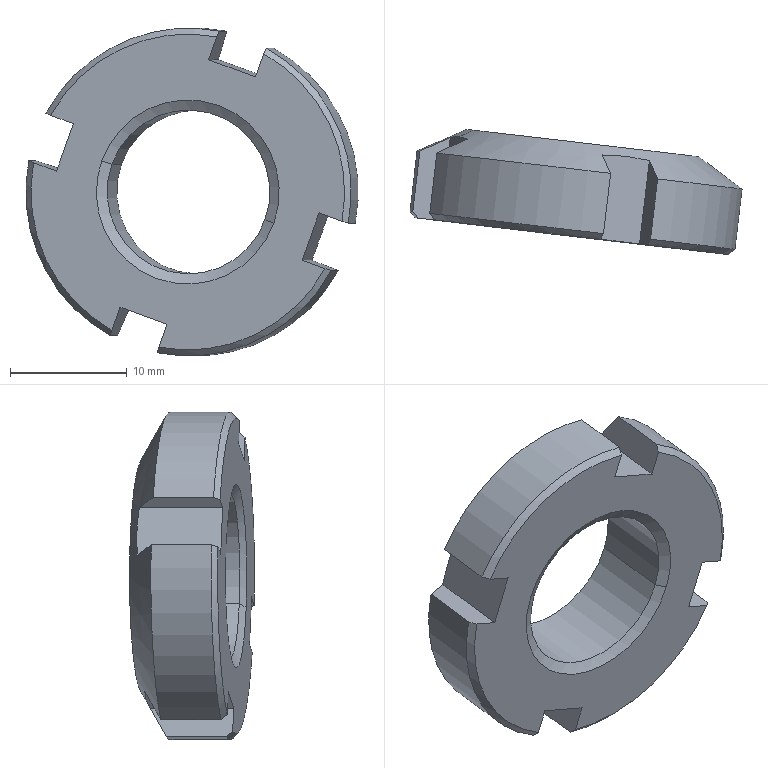Component | SolidWorks | 8TC-A17001-91-00UpperAndLowerPressAssembly-1_GB812RoundNutM14_1.5-1 | 1 solid | 30 faces | box 28.41 x 10.69 x 28 mm | volume 2997 mm3 | plane 14 | cone 10 | cylinder 6 | commonest cylinder face diameters 28 x4 14 x2 | material A3
STEP:
#1=CARTESIAN_POINT('',(-0.3344,-4.257,-1.954));
#2=VERTEX_POINT('',#1);
#3=CARTESIAN_POINT('',(0.1805,-4.318,-2.141));
#4=VERTEX_POINT('',#3);
#5=CARTESIAN_POINT('',(-0.07696,-4.287,-2.047));
#6=DIRECTION('',(-0.1167,-0.9932,0.));
#7=DIRECTION('',(0.9342,-0.1097,-0.3394));
#8=AXIS2_PLACEMENT_3D('',#5,#6,#7);
#9=CIRCLE('',#8,0.2756);
#10=EDGE_CURVE('',#2,#4,#9,.T.);
#11=ORIENTED_EDGE('',*,*,#10,.F.);
#12=CARTESIAN_POINT('',(-0.3686,-4.273,-1.942));
#13=VERTEX_POINT('',#12);
#14=CARTESIAN_POINT('',(-0.3344,-4.257,-1.954));
#15=DIRECTION('',(-0.8674,-0.4016,0.2939));
#16=VECTOR('',#15,39.37);
#17=LINE('',#14,#16);
#18=EDGE_CURVE('',#2,#13,#17,.T.);
#19=ORIENTED_EDGE('',*,*,#18,.T.);
#20=CARTESIAN_POINT('',(0.2101,-4.341,-2.152));
#21=VERTEX_POINT('',#20);
#22=CARTESIAN_POINT('',(-0.07926,-4.307,-2.047));
#23=DIRECTION('',(0.1167,0.9932,-0.));
#24=DIRECTION('',(0.9342,-0.1097,-0.3394));
#25=AXIS2_PLACEMENT_3D('',#22,#23,#24);
#26=CIRCLE('',#25,0.3097);
#27=EDGE_CURVE('',#21,#13,#26,.T.);
#28=ORIENTED_EDGE('',*,*,#27,.F.);
#29=CARTESIAN_POINT('',(0.1805,-4.318,-2.141));
#30=DIRECTION('',(0.7507,-0.5916,-0.2939));
#31=VECTOR('',#30,39.37);
#32=LINE('',#29,#31);
#33=EDGE_CURVE('',#4,#21,#32,.T.);
#34=ORIENTED_EDGE('',*,*,#33,.F.);
#35=EDGE_LOOP('',(#11,#19,#28,#34));
#36=FACE_OUTER_BOUND('',#35,.T.);
#37=CARTESIAN_POINT('',(-0.07696,-4.287,-2.047));
#38=DIRECTION('',(-0.1167,-0.9932,0.));
#39=DIRECTION('',(0.9342,-0.1097,-0.3394));
#40=AXIS2_PLACEMENT_3D('',#37,#38,#39);
#41=CONICAL_SURFACE('',#40,0.2756,1.047);
#42=ADVANCED_FACE('',(#36),#41,.F.);
#43=CARTESIAN_POINT('',(0.2126,-4.044,-2.141));
#44=VERTEX_POINT('',#43);
#45=CARTESIAN_POINT('',(-0.3023,-3.983,-1.954));
#46=VERTEX_POINT('',#45);
#47=CARTESIAN_POINT('',(-0.04481,-4.014,-2.047));
#48=DIRECTION('',(0.1167,0.9932,-0.));
#49=DIRECTION('',(0.9342,-0.1097,-0.3394));
#50=AXIS2_PLACEMENT_3D('',#47,#48,#49);
#51=CIRCLE('',#50,0.2756);
#52=EDGE_CURVE('',#44,#46,#51,.T.);
#53=ORIENTED_EDGE('',*,*,#52,.F.);
#54=CARTESIAN_POINT('',(0.2468,-4.028,-2.152));
#55=VERTEX_POINT('',#54);
#56=CARTESIAN_POINT('',(0.2468,-4.028,-2.152));
#57=DIRECTION('',(0.8674,0.4016,-0.2939));
#58=VECTOR('',#57,39.37);
#59=LINE('',#56,#58);
#60=EDGE_CURVE('',#44,#55,#59,.T.);
#61=ORIENTED_EDGE('',*,*,#60,.T.);
#62=CARTESIAN_POINT('',(-0.3318,-3.96,-1.942));
#63=VERTEX_POINT('',#62);
#64=CARTESIAN_POINT('',(-0.04251,-3.994,-2.047));
#65=DIRECTION('',(-0.1167,-0.9932,0.));
#66=DIRECTION('',(0.9342,-0.1097,-0.3394));
#67=AXIS2_PLACEMENT_3D('',#64,#65,#66);
#68=CIRCLE('',#67,0.3097);
#69=EDGE_CURVE('',#63,#55,#68,.T.);
#70=ORIENTED_EDGE('',*,*,#69,.F.);
#71=CARTESIAN_POINT('',(-0.3318,-3.96,-1.942));
#72=DIRECTION('',(-0.7507,0.5916,0.2939));
#73=VECTOR('',#72,39.37);
#74=LINE('',#71,#73);
#75=EDGE_CURVE('',#46,#63,#74,.T.);
#76=ORIENTED_EDGE('',*,*,#75,.F.);
#77=EDGE_LOOP('',(#53,#61,#70,#76));
#78=FACE_OUTER_BOUND('',#77,.T.);
#79=CARTESIAN_POINT('',(-0.04251,-3.994,-2.047));
#80=DIRECTION('',(0.1167,0.9932,-0.));
#81=DIRECTION('',(-0.9342,0.1097,0.3394));
#82=AXIS2_PLACEMENT_3D('',#79,#80,#81);
#83=CONICAL_SURFACE('',#82,0.3097,1.047);
#84=ADVANCED_FACE('',(#78),#83,.F.);
#85=CARTESIAN_POINT('',(-0.4103,-3.951,-1.914));
#86=VERTEX_POINT('',#85);
#87=CARTESIAN_POINT('',(0.3253,-4.037,-2.181));
#88=VERTEX_POINT('',#87);
#89=CARTESIAN_POINT('',(-0.04251,-3.994,-2.047));
#90=DIRECTION('',(0.1167,0.9932,-0.));
#91=DIRECTION('',(0.9342,-0.1097,-0.3394));
#92=AXIS2_PLACEMENT_3D('',#89,#90,#91);
#93=CIRCLE('',#92,0.3937);
#94=EDGE_CURVE('',#86,#88,#93,.T.);
#95=ORIENTED_EDGE('',*,*,#94,.F.);
#96=CARTESIAN_POINT('',(-0.459,-3.973,-1.897));
#97=VERTEX_POINT('',#96);
#98=CARTESIAN_POINT('',(-0.568,-4.024,-1.86));
#99=DIRECTION('',(-0.8674,-0.4015,0.2939));
#100=VECTOR('',#99,39.37);
#101=LINE('',#98,#100);
#102=EDGE_CURVE('',#86,#97,#101,.T.);
#103=ORIENTED_EDGE('',*,*,#102,.T.);
#104=CARTESIAN_POINT('',(-0.431,-3.981,-1.818));
#105=VERTEX_POINT('',#104);
#106=CARTESIAN_POINT('',(-0.431,-3.981,-1.818));
#107=CARTESIAN_POINT('',(-0.4401,-3.977,-1.844));
#108=CARTESIAN_POINT('',(-0.4494,-3.974,-1.87));
#109=CARTESIAN_POINT('',(-0.459,-3.973,-1.897));
#110=B_SPLINE_CURVE_WITH_KNOTS('',3,(#106,#107,#108,#109),.UNSPECIFIED.,.F.,.F.,(4,4),(0.002413,0.004566),.UNSPECIFIED.);
#111=EDGE_CURVE('',#105,#97,#110,.T.);
#112=ORIENTED_EDGE('',*,*,#111,.F.);
#113=CARTESIAN_POINT('',(-0.5334,-4.028,-1.783));
#114=VERTEX_POINT('',#113);
#115=CARTESIAN_POINT('',(-0.5334,-4.028,-1.783));
#116=CARTESIAN_POINT('',(-0.4993,-4.012,-1.794));
#117=CARTESIAN_POINT('',(-0.4651,-3.997,-1.806));
#118=CARTESIAN_POINT('',(-0.431,-3.981,-1.818));
#119=B_SPLINE_CURVE_WITH_KNOTS('',3,(#115,#116,#117,#118),.UNSPECIFIED.,.F.,.F.,(4,4),(0.005991,0.008982),.UNSPECIFIED.);
#120=EDGE_CURVE('',#114,#105,#119,.T.);
#121=ORIENTED_EDGE('',*,*,#120,.F.);
#122=CARTESIAN_POINT('',(0.0514,-4.097,-1.506));
#123=VERTEX_POINT('',#122);
#124=CARTESIAN_POINT('',(-0.05312,-4.084,-2.047));
#125=DIRECTION('',(-0.1167,-0.9932,0.));
#126=DIRECTION('',(0.9342,-0.1097,-0.3394));
#127=AXIS2_PLACEMENT_3D('',#124,#125,#126);
#128=CIRCLE('',#127,0.5512);
#129=EDGE_CURVE('',#123,#114,#128,.T.);
#130=ORIENTED_EDGE('',*,*,#129,.F.);
#131=CARTESIAN_POINT('',(0.02368,-4.035,-1.602));
#132=VERTEX_POINT('',#131);
#133=CARTESIAN_POINT('',(0.02368,-4.035,-1.602));
#134=CARTESIAN_POINT('',(0.03294,-4.055,-1.57));
#135=CARTESIAN_POINT('',(0.04217,-4.076,-1.538));
#136=CARTESIAN_POINT('',(0.0514,-4.097,-1.506));
#137=B_SPLINE_CURVE_WITH_KNOTS('',3,(#133,#134,#135,#136),.UNSPECIFIED.,.F.,.F.,(4,4),(0.006116,0.009107),.UNSPECIFIED.);
#138=EDGE_CURVE('',#132,#123,#137,.T.);
#139=ORIENTED_EDGE('',*,*,#138,.F.);
#140=CARTESIAN_POINT('',(0.1818,-4.053,-1.66));
#141=VERTEX_POINT('',#140);
#142=CARTESIAN_POINT('',(0.1818,-4.053,-1.66));
#143=CARTESIAN_POINT('',(0.156,-4.047,-1.65));
#144=CARTESIAN_POINT('',(0.1299,-4.043,-1.641));
#145=CARTESIAN_POINT('',(0.09038,-4.038,-1.627));
#146=CARTESIAN_POINT('',(0.07712,-4.037,-1.622));
#147=CARTESIAN_POINT('',(0.05046,-4.035,-1.612));
#148=CARTESIAN_POINT('',(0.03703,-4.035,-1.607));
#149=CARTESIAN_POINT('',(0.02368,-4.035,-1.602));
#150=B_SPLINE_CURVE_WITH_KNOTS('',3,(#142,#143,#144,#145,#146,#147,#148,#149),.UNSPECIFIED.,.F.,.F.,(4,2,2,4),(0.002413,0.004558,0.005631,0.006704),.UNSPECIFIED.);
#151=EDGE_CURVE('',#141,#132,#150,.T.);
#152=ORIENTED_EDGE('',*,*,#151,.F.);
#153=CARTESIAN_POINT('',(0.2096,-4.115,-1.564));
#154=VERTEX_POINT('',#153);
#155=CARTESIAN_POINT('',(0.2096,-4.115,-1.564));
#156=CARTESIAN_POINT('',(0.2003,-4.095,-1.596));
#157=CARTESIAN_POINT('',(0.1911,-4.074,-1.628));
#158=CARTESIAN_POINT('',(0.1818,-4.053,-1.66));
#159=B_SPLINE_CURVE_WITH_KNOTS('',3,(#155,#156,#157,#158),.UNSPECIFIED.,.F.,.F.,(4,4),(0.003725,0.006717),.UNSPECIFIED.);
#160=EDGE_CURVE('',#154,#141,#159,.T.);
#161=ORIENTED_EDGE('',*,*,#160,.F.);
#162=CARTESIAN_POINT('',(0.4842,-4.147,-2.152));
#163=VERTEX_POINT('',#162);
#164=CARTESIAN_POINT('',(-0.05312,-4.084,-2.047));
#165=DIRECTION('',(-0.1167,-0.9932,0.));
#166=DIRECTION('',(0.9342,-0.1097,-0.3394));
#167=AXIS2_PLACEMENT_3D('',#164,#165,#166);
#168=CIRCLE('',#167,0.5512);
#169=EDGE_CURVE('',#163,#154,#168,.T.);
#170=ORIENTED_EDGE('',*,*,#169,.F.);
#171=CARTESIAN_POINT('',(0.3954,-4.078,-2.118));
#172=VERTEX_POINT('',#171);
#173=CARTESIAN_POINT('',(0.3954,-4.078,-2.118));
#174=CARTESIAN_POINT('',(0.425,-4.101,-2.129));
#175=CARTESIAN_POINT('',(0.4546,-4.124,-2.141));
#176=CARTESIAN_POINT('',(0.4842,-4.147,-2.152));
#177=B_SPLINE_CURVE_WITH_KNOTS('',3,(#173,#174,#175,#176),.UNSPECIFIED.,.F.,.F.,(4,4),(0.006116,0.009107),.UNSPECIFIED.);
#178=EDGE_CURVE('',#172,#163,#177,.T.);
#179=ORIENTED_EDGE('',*,*,#178,.F.);
#180=CARTESIAN_POINT('',(0.3674,-4.07,-2.197));
#181=VERTEX_POINT('',#180);
#182=CARTESIAN_POINT('',(0.3674,-4.07,-2.197));
#183=CARTESIAN_POINT('',(0.3769,-4.072,-2.171));
#184=CARTESIAN_POINT('',(0.3863,-4.074,-2.144));
#185=CARTESIAN_POINT('',(0.3954,-4.078,-2.118));
#186=B_SPLINE_CURVE_WITH_KNOTS('',3,(#182,#183,#184,#185),.UNSPECIFIED.,.F.,.F.,(4,4),(0.01138,0.01353),.UNSPECIFIED.);
#187=EDGE_CURVE('',#181,#172,#186,.T.);
#188=ORIENTED_EDGE('',*,*,#187,.F.);
#189=CARTESIAN_POINT('',(0.4618,-4.145,-2.234));
#190=DIRECTION('',(0.7507,-0.5916,-0.2939));
#191=VECTOR('',#190,39.37);
#192=LINE('',#189,#191);
#193=EDGE_CURVE('',#88,#181,#192,.T.);
#194=ORIENTED_EDGE('',*,*,#193,.F.);
#195=EDGE_LOOP('',(#95,#103,#112,#121,#130,#139,#152,#161,#170,#179,#188,#194));
#196=FACE_OUTER_BOUND('',#195,.T.);
#197=CARTESIAN_POINT('',(-0.05312,-4.084,-2.047));
#198=DIRECTION('',(-0.1167,-0.9932,0.));
#199=DIRECTION('',(0.9342,-0.1097,-0.3394));
#200=AXIS2_PLACEMENT_3D('',#197,#198,#199);
#201=CONICAL_SURFACE('',#200,0.5512,1.047);
#202=ADVANCED_FACE('',(#196),#201,.T.);
#203=ORIENTED_EDGE('',*,*,#10,.T.);
#204=CARTESIAN_POINT('',(0.1782,-4.337,-2.141));
#205=DIRECTION('',(0.1167,0.9932,-0.));
#206=VECTOR('',#205,39.37);
#207=LINE('',#204,#206);
#208=EDGE_CURVE('',#4,#44,#207,.T.);
#209=ORIENTED_EDGE('',*,*,#208,.T.);
#210=ORIENTED_EDGE('',*,*,#52,.T.);
#211=CARTESIAN_POINT('',(-0.3367,-4.277,-1.954));
#212=DIRECTION('',(0.1167,0.9932,-0.));
#213=VECTOR('',#212,39.37);
#214=LINE('',#211,#213);
#215=EDGE_CURVE('',#2,#46,#214,.T.);
#216=ORIENTED_EDGE('',*,*,#215,.F.);
#217=EDGE_LOOP('',(#203,#209,#210,#216));
#218=FACE_OUTER_BOUND('',#217,.T.);
#219=CARTESIAN_POINT('',(-0.07926,-4.307,-2.047));
#220=DIRECTION('',(0.1167,0.9932,-0.));
#221=DIRECTION('',(-0.9342,0.1097,0.3394));
#222=AXIS2_PLACEMENT_3D('',#219,#220,#221);
#223=CYLINDRICAL_SURFACE('',#222,0.2756);
#224=ADVANCED_FACE('',(#218),#223,.F.);
#225=CARTESIAN_POINT('',(0.1857,-4.318,-1.564));
#226=VERTEX_POINT('',#225);
#227=CARTESIAN_POINT('',(0.4604,-4.35,-2.152));
#228=VERTEX_POINT('',#227);
#229=CARTESIAN_POINT('',(-0.07696,-4.287,-2.047));
#230=DIRECTION('',(0.1167,0.9932,-0.));
#231=DIRECTION('',(0.9342,-0.1097,-0.3394));
#232=AXIS2_PLACEMENT_3D('',#229,#230,#231);
#233=CIRCLE('',#232,0.5512);
#234=EDGE_CURVE('',#226,#228,#233,.T.);
#235=ORIENTED_EDGE('',*,*,#234,.T.);
#236=CARTESIAN_POINT('',(0.4948,-4.057,-2.152));
#237=DIRECTION('',(-0.1167,-0.9932,0.));
#238=VECTOR('',#237,39.37);
#239=LINE('',#236,#238);
#240=EDGE_CURVE('',#163,#228,#239,.T.);
#241=ORIENTED_EDGE('',*,*,#240,.F.);
#242=ORIENTED_EDGE('',*,*,#169,.T.);
#243=CARTESIAN_POINT('',(0.2202,-4.025,-1.564));
#244=DIRECTION('',(-0.1167,-0.9932,0.));
#245=VECTOR('',#244,39.37);
#246=LINE('',#243,#245);
#247=EDGE_CURVE('',#154,#226,#246,.T.);
#248=ORIENTED_EDGE('',*,*,#247,.T.);
#249=EDGE_LOOP('',(#235,#241,#242,#248));
#250=FACE_OUTER_BOUND('',#249,.T.);
#251=CARTESIAN_POINT('',(-0.07926,-4.307,-2.047));
#252=DIRECTION('',(0.1167,0.9932,-0.));
#253=DIRECTION('',(-0.9342,0.1097,0.3394));
#254=AXIS2_PLACEMENT_3D('',#251,#252,#253);
#255=CYLINDRICAL_SURFACE('',#254,0.5512);
#256=ADVANCED_FACE('',(#250),#255,.T.);
#257=CARTESIAN_POINT('',(0.4395,-4.368,-2.146));
#258=VERTEX_POINT('',#257);
#259=CARTESIAN_POINT('',(0.4604,-4.35,-2.152));
#260=CARTESIAN_POINT('',(0.4534,-4.356,-2.15));
#261=CARTESIAN_POINT('',(0.4464,-4.362,-2.148));
#262=CARTESIAN_POINT('',(0.4395,-4.368,-2.146));
#263=B_SPLINE_CURVE_WITH_KNOTS('',3,(#259,#260,#261,#262),.UNSPECIFIED.,.F.,.F.,(4,4),(0.004508,0.005219),.UNSPECIFIED.);
#264=EDGE_CURVE('',#228,#258,#263,.T.);
#265=ORIENTED_EDGE('',*,*,#264,.F.);
#266=ORIENTED_EDGE('',*,*,#234,.F.);
#267=CARTESIAN_POINT('',(0.1767,-4.337,-1.582));
#268=VERTEX_POINT('',#267);
#269=CARTESIAN_POINT('',(0.1767,-4.337,-1.582));
#270=CARTESIAN_POINT('',(0.1797,-4.331,-1.576));
#271=CARTESIAN_POINT('',(0.1827,-4.324,-1.57));
#272=CARTESIAN_POINT('',(0.1857,-4.318,-1.564));
#273=B_SPLINE_CURVE_WITH_KNOTS('',3,(#269,#270,#271,#272),.UNSPECIFIED.,.F.,.F.,(4,4),(0.00461,0.005321),.UNSPECIFIED.);
#274=EDGE_CURVE('',#268,#226,#273,.T.);
#275=ORIENTED_EDGE('',*,*,#274,.F.);
#276=CARTESIAN_POINT('',(-0.07926,-4.307,-2.047));
#277=DIRECTION('',(-0.1167,-0.9932,0.));
#278=DIRECTION('',(0.9342,-0.1097,-0.3394));
#279=AXIS2_PLACEMENT_3D('',#276,#277,#278);
#280=CIRCLE('',#279,0.5315);
#281=EDGE_CURVE('',#258,#268,#280,.T.);
#282=ORIENTED_EDGE('',*,*,#281,.F.);
#283=EDGE_LOOP('',(#265,#266,#275,#282));
#284=FACE_OUTER_BOUND('',#283,.T.);
#285=CARTESIAN_POINT('',(-0.07926,-4.307,-2.047));
#286=DIRECTION('',(0.1167,0.9932,-0.));
#287=DIRECTION('',(-0.9342,0.1097,0.3394));
#288=AXIS2_PLACEMENT_3D('',#285,#286,#287);
#289=CONICAL_SURFACE('',#288,0.5315,0.7854);
#290=ADVANCED_FACE('',(#284),#289,.T.);
#291=CARTESIAN_POINT('',(-0.5572,-4.231,-1.783));
#292=VERTEX_POINT('',#291);
#293=CARTESIAN_POINT('',(0.02755,-4.3,-1.506));
#294=VERTEX_POINT('',#293);
#295=CARTESIAN_POINT('',(-0.07696,-4.287,-2.047));
#296=DIRECTION('',(0.1167,0.9932,-0.));
#297=DIRECTION('',(0.9342,-0.1097,-0.3394));
#298=AXIS2_PLACEMENT_3D('',#295,#296,#297);
#299=CIRCLE('',#298,0.5512);
#300=EDGE_CURVE('',#292,#294,#299,.T.);
#301=ORIENTED_EDGE('',*,*,#300,.T.);
#302=CARTESIAN_POINT('',(0.062,-4.006,-1.506));
#303=DIRECTION('',(-0.1167,-0.9932,0.));
#304=VECTOR('',#303,39.37);
#305=LINE('',#302,#304);
#306=EDGE_CURVE('',#123,#294,#305,.T.);
#307=ORIENTED_EDGE('',*,*,#306,.F.);
#308=ORIENTED_EDGE('',*,*,#129,.T.);
#309=CARTESIAN_POINT('',(-0.5228,-3.938,-1.783));
#310=DIRECTION('',(-0.1167,-0.9932,0.));
#311=VECTOR('',#310,39.37);
#312=LINE('',#309,#311);
#313=EDGE_CURVE('',#114,#292,#312,.T.);
#314=ORIENTED_EDGE('',*,*,#313,.T.);
#315=EDGE_LOOP('',(#301,#307,#308,#314));
#316=FACE_OUTER_BOUND('',#315,.T.);
#317=CARTESIAN_POINT('',(-0.07926,-4.307,-2.047));
#318=DIRECTION('',(0.1167,0.9932,-0.));
#319=DIRECTION('',(-0.9342,0.1097,0.3394));
#320=AXIS2_PLACEMENT_3D('',#317,#318,#319);
#321=CYLINDRICAL_SURFACE('',#320,0.5512);
#322=ADVANCED_FACE('',(#316),#321,.T.);
#323=CARTESIAN_POINT('',(0.01854,-4.318,-1.525));
#324=VERTEX_POINT('',#323);
#325=CARTESIAN_POINT('',(0.02755,-4.3,-1.506));
#326=CARTESIAN_POINT('',(0.02455,-4.306,-1.512));
#327=CARTESIAN_POINT('',(0.02154,-4.312,-1.519));
#328=CARTESIAN_POINT('',(0.01854,-4.318,-1.525));
#329=B_SPLINE_CURVE_WITH_KNOTS('',3,(#325,#326,#327,#328),.UNSPECIFIED.,.F.,.F.,(4,4),(0.004508,0.005219),.UNSPECIFIED.);
#330=EDGE_CURVE('',#294,#324,#329,.T.);
#331=ORIENTED_EDGE('',*,*,#330,.F.);
#332=ORIENTED_EDGE('',*,*,#300,.F.);
#333=CARTESIAN_POINT('',(-0.5409,-4.253,-1.79));
#334=VERTEX_POINT('',#333);
#335=CARTESIAN_POINT('',(-0.5409,-4.253,-1.79));
#336=CARTESIAN_POINT('',(-0.5464,-4.245,-1.787));
#337=CARTESIAN_POINT('',(-0.5518,-4.238,-1.785));
#338=CARTESIAN_POINT('',(-0.5572,-4.231,-1.783));
#339=B_SPLINE_CURVE_WITH_KNOTS('',3,(#335,#336,#337,#338),.UNSPECIFIED.,.F.,.F.,(4,4),(0.00461,0.005321),.UNSPECIFIED.);
#340=EDGE_CURVE('',#334,#292,#339,.T.);
#341=ORIENTED_EDGE('',*,*,#340,.F.);
#342=CARTESIAN_POINT('',(-0.07926,-4.307,-2.047));
#343=DIRECTION('',(-0.1167,-0.9932,0.));
#344=DIRECTION('',(0.9342,-0.1097,-0.3394));
#345=AXIS2_PLACEMENT_3D('',#342,#343,#344);
#346=CIRCLE('',#345,0.5315);
#347=EDGE_CURVE('',#324,#334,#346,.T.);
#348=ORIENTED_EDGE('',*,*,#347,.F.);
#349=EDGE_LOOP('',(#331,#332,#341,#348));
#350=FACE_OUTER_BOUND('',#349,.T.);
#351=CARTESIAN_POINT('',(-0.07926,-4.307,-2.047));
#352=DIRECTION('',(0.1167,0.9932,-0.));
#353=DIRECTION('',(-0.9342,0.1097,0.3394));
#354=AXIS2_PLACEMENT_3D('',#351,#352,#353);
#355=CONICAL_SURFACE('',#354,0.5315,0.7854);
#356=ADVANCED_FACE('',(#350),#355,.T.);
#357=CARTESIAN_POINT('',(-0.3396,-4.256,-2.531));
#358=VERTEX_POINT('',#357);
#359=CARTESIAN_POINT('',(-0.6143,-4.224,-1.942));
#360=VERTEX_POINT('',#359);
#361=CARTESIAN_POINT('',(-0.07696,-4.287,-2.047));
#362=DIRECTION('',(0.1167,0.9932,-0.));
#363=DIRECTION('',(0.9342,-0.1097,-0.3394));
#364=AXIS2_PLACEMENT_3D('',#361,#362,#363);
#365=CIRCLE('',#364,0.5512);
#366=EDGE_CURVE('',#358,#360,#365,.T.);
#367=ORIENTED_EDGE('',*,*,#366,.T.);
#368=CARTESIAN_POINT('',(-0.5905,-4.021,-1.942));
#369=VERTEX_POINT('',#368);
#370=CARTESIAN_POINT('',(-0.5799,-3.931,-1.942));
#371=DIRECTION('',(-0.1167,-0.9932,0.));
#372=VECTOR('',#371,39.37);
#373=LINE('',#370,#372);
#374=EDGE_CURVE('',#369,#360,#373,.T.);
#375=ORIENTED_EDGE('',*,*,#374,.F.);
#376=CARTESIAN_POINT('',(-0.3158,-4.053,-2.531));
#377=VERTEX_POINT('',#376);
#378=CARTESIAN_POINT('',(-0.05312,-4.084,-2.047));
#379=DIRECTION('',(-0.1167,-0.9932,0.));
#380=DIRECTION('',(0.9342,-0.1097,-0.3394));
#381=AXIS2_PLACEMENT_3D('',#378,#379,#380);
#382=CIRCLE('',#381,0.5512);
#383=EDGE_CURVE('',#369,#377,#382,.T.);
#384=ORIENTED_EDGE('',*,*,#383,.T.);
#385=CARTESIAN_POINT('',(-0.3052,-3.963,-2.531));
#386=DIRECTION('',(-0.1167,-0.9932,0.));
#387=VECTOR('',#386,39.37);
#388=LINE('',#385,#387);
#389=EDGE_CURVE('',#377,#358,#388,.T.);
#390=ORIENTED_EDGE('',*,*,#389,.T.);
#391=EDGE_LOOP('',(#367,#375,#384,#390));
#392=FACE_OUTER_BOUND('',#391,.T.);
#393=CARTESIAN_POINT('',(-0.07926,-4.307,-2.047));
#394=DIRECTION('',(0.1167,0.9932,-0.));
#395=DIRECTION('',(-0.9342,0.1097,0.3394));
#396=AXIS2_PLACEMENT_3D('',#393,#394,#395);
#397=CYLINDRICAL_SURFACE('',#396,0.5512);
#398=ADVANCED_FACE('',(#392),#397,.T.);
#399=CARTESIAN_POINT('',(-0.598,-4.246,-1.949));
#400=VERTEX_POINT('',#399);
#401=CARTESIAN_POINT('',(-0.6143,-4.224,-1.942));
#402=CARTESIAN_POINT('',(-0.6089,-4.231,-1.944));
#403=CARTESIAN_POINT('',(-0.6034,-4.239,-1.947));
#404=CARTESIAN_POINT('',(-0.598,-4.246,-1.949));
#405=B_SPLINE_CURVE_WITH_KNOTS('',3,(#401,#402,#403,#404),.UNSPECIFIED.,.F.,.F.,(4,4),(0.004508,0.005219),.UNSPECIFIED.);
#406=EDGE_CURVE('',#360,#400,#405,.T.);
#407=ORIENTED_EDGE('',*,*,#406,.F.);
#408=ORIENTED_EDGE('',*,*,#366,.F.);
#409=CARTESIAN_POINT('',(-0.3352,-4.277,-2.512));
#410=VERTEX_POINT('',#409);
#411=CARTESIAN_POINT('',(-0.3352,-4.277,-2.512));
#412=CARTESIAN_POINT('',(-0.3367,-4.27,-2.518));
#413=CARTESIAN_POINT('',(-0.3382,-4.263,-2.525));
#414=CARTESIAN_POINT('',(-0.3396,-4.256,-2.531));
#415=B_SPLINE_CURVE_WITH_KNOTS('',3,(#411,#412,#413,#414),.UNSPECIFIED.,.F.,.F.,(4,4),(0.00461,0.005321),.UNSPECIFIED.);
#416=EDGE_CURVE('',#410,#358,#415,.T.);
#417=ORIENTED_EDGE('',*,*,#416,.F.);
#418=CARTESIAN_POINT('',(-0.07926,-4.307,-2.047));
#419=DIRECTION('',(-0.1167,-0.9932,0.));
#420=DIRECTION('',(0.9342,-0.1097,-0.3394));
#421=AXIS2_PLACEMENT_3D('',#418,#419,#420);
#422=CIRCLE('',#421,0.5315);
#423=EDGE_CURVE('',#400,#410,#422,.T.);
#424=ORIENTED_EDGE('',*,*,#423,.F.);
#425=EDGE_LOOP('',(#407,#408,#417,#424));
#426=FACE_OUTER_BOUND('',#425,.T.);
#427=CARTESIAN_POINT('',(-0.07926,-4.307,-2.047));
#428=DIRECTION('',(0.1167,0.9932,-0.));
#429=DIRECTION('',(-0.9342,0.1097,0.3394));
#430=AXIS2_PLACEMENT_3D('',#427,#428,#429);
#431=CONICAL_SURFACE('',#430,0.5315,0.7854);
#432=ADVANCED_FACE('',(#426),#431,.T.);
#433=ORIENTED_EDGE('',*,*,#27,.T.);
#434=CARTESIAN_POINT('',(-0.07926,-4.307,-2.047));
#435=DIRECTION('',(0.1167,0.9932,-0.));
#436=DIRECTION('',(0.9342,-0.1097,-0.3394));
#437=AXIS2_PLACEMENT_3D('',#434,#435,#436);
#438=CIRCLE('',#437,0.3097);
#439=EDGE_CURVE('',#13,#21,#438,.T.);
#440=ORIENTED_EDGE('',*,*,#439,.T.);
#441=EDGE_LOOP('',(#433,#440));
#442=FACE_BOUND('',#441,.T.);
#443=CARTESIAN_POINT('',(0.3625,-4.359,-2.118));
#444=VERTEX_POINT('',#443);
#445=CARTESIAN_POINT('',(0.3625,-4.359,-2.118));
#446=DIRECTION('',(-0.9342,0.1097,0.3394));
#447=VECTOR('',#446,39.37);
#448=LINE('',#445,#447);
#449=EDGE_CURVE('',#258,#444,#448,.T.);
#450=ORIENTED_EDGE('',*,*,#449,.F.);
#451=ORIENTED_EDGE('',*,*,#281,.T.);
#452=CARTESIAN_POINT('',(0.1489,-4.334,-1.66));
#453=VERTEX_POINT('',#452);
#454=CARTESIAN_POINT('',(0.1489,-4.334,-1.66));
#455=DIRECTION('',(0.3371,-0.0396,0.9406));
#456=VECTOR('',#455,39.37);
#457=LINE('',#454,#456);
#458=EDGE_CURVE('',#453,#268,#457,.T.);
#459=ORIENTED_EDGE('',*,*,#458,.F.);
#460=CARTESIAN_POINT('',(-0.009248,-4.315,-1.602));
#461=VERTEX_POINT('',#460);
#462=CARTESIAN_POINT('',(0.1489,-4.334,-1.66));
#463=DIRECTION('',(0.9342,-0.1097,-0.3394));
#464=VECTOR('',#463,39.37);
#465=LINE('',#462,#464);
#466=EDGE_CURVE('',#461,#453,#465,.T.);
#467=ORIENTED_EDGE('',*,*,#466,.F.);
#468=CARTESIAN_POINT('',(-0.009248,-4.315,-1.602));
#469=DIRECTION('',(-0.3371,0.0396,-0.9406));
#470=VECTOR('',#469,39.37);
#471=LINE('',#468,#470);
#472=EDGE_CURVE('',#324,#461,#471,.T.);
#473=ORIENTED_EDGE('',*,*,#472,.F.);
#474=ORIENTED_EDGE('',*,*,#347,.T.);
#475=CARTESIAN_POINT('',(-0.4639,-4.262,-1.818));
#476=VERTEX_POINT('',#475);
#477=CARTESIAN_POINT('',(-0.4639,-4.262,-1.818));
#478=DIRECTION('',(-0.9342,0.1097,0.3394));
#479=VECTOR('',#478,39.37);
#480=LINE('',#477,#479);
#481=EDGE_CURVE('',#476,#334,#480,.T.);
#482=ORIENTED_EDGE('',*,*,#481,.F.);
#483=CARTESIAN_POINT('',(-0.521,-4.255,-1.977));
#484=VERTEX_POINT('',#483);
#485=CARTESIAN_POINT('',(-0.4639,-4.262,-1.818));
#486=DIRECTION('',(0.3371,-0.0396,0.9406));
#487=VECTOR('',#486,39.37);
#488=LINE('',#485,#487);
#489=EDGE_CURVE('',#484,#476,#488,.T.);
#490=ORIENTED_EDGE('',*,*,#489,.F.);
#491=CARTESIAN_POINT('',(-0.521,-4.255,-1.977));
#492=DIRECTION('',(0.9342,-0.1097,-0.3394));
#493=VECTOR('',#492,39.37);
#494=LINE('',#491,#493);
#495=EDGE_CURVE('',#400,#484,#494,.T.);
#496=ORIENTED_EDGE('',*,*,#495,.F.);
#497=ORIENTED_EDGE('',*,*,#423,.T.);
#498=CARTESIAN_POINT('',(-0.3074,-4.28,-2.435));
#499=VERTEX_POINT('',#498);
#500=CARTESIAN_POINT('',(-0.3074,-4.28,-2.435));
#501=DIRECTION('',(-0.3371,0.0396,-0.9406));
#502=VECTOR('',#501,39.37);
#503=LINE('',#500,#502);
#504=EDGE_CURVE('',#499,#410,#503,.T.);
#505=ORIENTED_EDGE('',*,*,#504,.F.);
#506=CARTESIAN_POINT('',(-0.1493,-4.299,-2.492));
#507=VERTEX_POINT('',#506);
#508=CARTESIAN_POINT('',(-0.3074,-4.28,-2.435));
#509=DIRECTION('',(-0.9342,0.1097,0.3394));
#510=VECTOR('',#509,39.37);
#511=LINE('',#508,#510);
#512=EDGE_CURVE('',#507,#499,#511,.T.);
#513=ORIENTED_EDGE('',*,*,#512,.F.);
#514=CARTESIAN_POINT('',(-0.1771,-4.295,-2.57));
#515=VERTEX_POINT('',#514);
#516=CARTESIAN_POINT('',(-0.1493,-4.299,-2.492));
#517=DIRECTION('',(0.3371,-0.0396,0.9406));
#518=VECTOR('',#517,39.37);
#519=LINE('',#516,#518);
#520=EDGE_CURVE('',#515,#507,#519,.T.);
#521=ORIENTED_EDGE('',*,*,#520,.F.);
#522=CARTESIAN_POINT('',(0.3824,-4.361,-2.305));
#523=VERTEX_POINT('',#522);
#524=CARTESIAN_POINT('',(-0.07926,-4.307,-2.047));
#525=DIRECTION('',(-0.1167,-0.9932,0.));
#526=DIRECTION('',(0.9342,-0.1097,-0.3394));
#527=AXIS2_PLACEMENT_3D('',#524,#525,#526);
#528=CIRCLE('',#527,0.5315);
#529=EDGE_CURVE('',#515,#523,#528,.T.);
#530=ORIENTED_EDGE('',*,*,#529,.T.);
#531=CARTESIAN_POINT('',(0.3054,-4.352,-2.277));
#532=VERTEX_POINT('',#531);
#533=CARTESIAN_POINT('',(0.3054,-4.352,-2.277));
#534=DIRECTION('',(0.9342,-0.1097,-0.3394));
#535=VECTOR('',#534,39.37);
#536=LINE('',#533,#535);
#537=EDGE_CURVE('',#532,#523,#536,.T.);
#538=ORIENTED_EDGE('',*,*,#537,.F.);
#539=CARTESIAN_POINT('',(0.3054,-4.352,-2.277));
#540=DIRECTION('',(-0.3371,0.0396,-0.9406));
#541=VECTOR('',#540,39.37);
#542=LINE('',#539,#541);
#543=EDGE_CURVE('',#444,#532,#542,.T.);
#544=ORIENTED_EDGE('',*,*,#543,.F.);
#545=EDGE_LOOP('',(#450,#451,#459,#467,#473,#474,#482,#490,#496,#497,#505,#513,#521,#530,#538,#544));
#546=FACE_OUTER_BOUND('',#545,.T.);
#547=CARTESIAN_POINT('',(-0.07926,-4.307,-2.047));
#548=DIRECTION('',(-0.1167,-0.9932,0.));
#549=DIRECTION('',(0.9342,-0.1097,-0.3394));
#550=AXIS2_PLACEMENT_3D('',#547,#548,#549);
#551=PLANE('',#550);
#552=ADVANCED_FACE('',(#442,#546),#551,.T.);
#553=ORIENTED_EDGE('',*,*,#69,.T.);
#554=CARTESIAN_POINT('',(-0.04251,-3.994,-2.047));
#555=DIRECTION('',(-0.1167,-0.9932,0.));
#556=DIRECTION('',(0.9342,-0.1097,-0.3394));
#557=AXIS2_PLACEMENT_3D('',#554,#555,#556);
#558=CIRCLE('',#557,0.3097);
#559=EDGE_CURVE('',#55,#63,#558,.T.);
#560=ORIENTED_EDGE('',*,*,#559,.T.);
#561=EDGE_LOOP('',(#553,#560));
#562=FACE_BOUND('',#561,.T.);
#563=CARTESIAN_POINT('',(-0.04251,-3.994,-2.047));
#564=DIRECTION('',(0.1167,0.9932,-0.));
#565=DIRECTION('',(0.9342,-0.1097,-0.3394));
#566=AXIS2_PLACEMENT_3D('',#563,#564,#565);
#567=CIRCLE('',#566,0.3937);
#568=EDGE_CURVE('',#88,#86,#567,.T.);
#569=ORIENTED_EDGE('',*,*,#568,.T.);
#570=ORIENTED_EDGE('',*,*,#94,.T.);
#571=EDGE_LOOP('',(#569,#570));
#572=FACE_OUTER_BOUND('',#571,.T.);
#573=CARTESIAN_POINT('',(-0.04251,-3.994,-2.047));
#574=DIRECTION('',(-0.1167,-0.9932,0.));
#575=DIRECTION('',(0.9342,-0.1097,-0.3394));
#576=AXIS2_PLACEMENT_3D('',#573,#574,#575);
#577=PLANE('',#576);
#578=ADVANCED_FACE('',(#562,#572),#577,.F.);
#579=CARTESIAN_POINT('',(-0.1576,-4.072,-2.588));
#580=VERTEX_POINT('',#579);
#581=CARTESIAN_POINT('',(0.4272,-4.141,-2.312));
#582=VERTEX_POINT('',#581);
#583=CARTESIAN_POINT('',(-0.05312,-4.084,-2.047));
#584=DIRECTION('',(-0.1167,-0.9932,0.));
#585=DIRECTION('',(0.9342,-0.1097,-0.3394));
#586=AXIS2_PLACEMENT_3D('',#583,#584,#585);
#587=CIRCLE('',#586,0.5512);
#588=EDGE_CURVE('',#580,#582,#587,.T.);
#589=ORIENTED_EDGE('',*,*,#588,.T.);
#590=CARTESIAN_POINT('',(0.4033,-4.344,-2.312));
#591=VERTEX_POINT('',#590);
#592=CARTESIAN_POINT('',(0.4378,-4.05,-2.312));
#593=DIRECTION('',(-0.1167,-0.9932,0.));
#594=VECTOR('',#593,39.37);
#595=LINE('',#592,#594);
#596=EDGE_CURVE('',#582,#591,#595,.T.);
#597=ORIENTED_EDGE('',*,*,#596,.T.);
#598=CARTESIAN_POINT('',(-0.1815,-4.275,-2.588));
#599=VERTEX_POINT('',#598);
#600=CARTESIAN_POINT('',(-0.07696,-4.287,-2.047));
#601=DIRECTION('',(0.1167,0.9932,-0.));
#602=DIRECTION('',(0.9342,-0.1097,-0.3394));
#603=AXIS2_PLACEMENT_3D('',#600,#601,#602);
#604=CIRCLE('',#603,0.5512);
#605=EDGE_CURVE('',#591,#599,#604,.T.);
#606=ORIENTED_EDGE('',*,*,#605,.T.);
#607=CARTESIAN_POINT('',(-0.147,-3.982,-2.588));
#608=DIRECTION('',(-0.1167,-0.9932,0.));
#609=VECTOR('',#608,39.37);
#610=LINE('',#607,#609);
#611=EDGE_CURVE('',#580,#599,#610,.T.);
#612=ORIENTED_EDGE('',*,*,#611,.F.);
#613=EDGE_LOOP('',(#589,#597,#606,#612));
#614=FACE_OUTER_BOUND('',#613,.T.);
#615=CARTESIAN_POINT('',(-0.07926,-4.307,-2.047));
#616=DIRECTION('',(0.1167,0.9932,-0.));
#617=DIRECTION('',(-0.9342,0.1097,0.3394));
#618=AXIS2_PLACEMENT_3D('',#615,#616,#617);
#619=CYLINDRICAL_SURFACE('',#618,0.5512);
#620=ADVANCED_FACE('',(#614),#619,.T.);
#621=ORIENTED_EDGE('',*,*,#208,.F.);
#622=CARTESIAN_POINT('',(-0.07696,-4.287,-2.047));
#623=DIRECTION('',(-0.1167,-0.9932,0.));
#624=DIRECTION('',(0.9342,-0.1097,-0.3394));
#625=AXIS2_PLACEMENT_3D('',#622,#623,#624);
#626=CIRCLE('',#625,0.2756);
#627=EDGE_CURVE('',#4,#2,#626,.T.);
#628=ORIENTED_EDGE('',*,*,#627,.T.);
#629=ORIENTED_EDGE('',*,*,#215,.T.);
#630=CARTESIAN_POINT('',(-0.04481,-4.014,-2.047));
#631=DIRECTION('',(0.1167,0.9932,-0.));
#632=DIRECTION('',(0.9342,-0.1097,-0.3394));
#633=AXIS2_PLACEMENT_3D('',#630,#631,#632);
#634=CIRCLE('',#633,0.2756);
#635=EDGE_CURVE('',#46,#44,#634,.T.);
#636=ORIENTED_EDGE('',*,*,#635,.T.);
#637=EDGE_LOOP('',(#621,#628,#629,#636));
#638=FACE_OUTER_BOUND('',#637,.T.);
#639=CARTESIAN_POINT('',(-0.07926,-4.307,-2.047));
#640=DIRECTION('',(0.1167,0.9932,-0.));
#641=DIRECTION('',(-0.9342,0.1097,0.3394));
#642=AXIS2_PLACEMENT_3D('',#639,#640,#641);
#643=CYLINDRICAL_SURFACE('',#642,0.2756);
#644=ADVANCED_FACE('',(#638),#643,.F.);
#645=CARTESIAN_POINT('',(0.3824,-4.361,-2.305));
#646=CARTESIAN_POINT('',(0.3894,-4.355,-2.307));
#647=CARTESIAN_POINT('',(0.3963,-4.35,-2.309));
#648=CARTESIAN_POINT('',(0.4033,-4.344,-2.312));
#649=B_SPLINE_CURVE_WITH_KNOTS('',3,(#645,#646,#647,#648),.UNSPECIFIED.,.F.,.F.,(4,4),(0.00461,0.005321),.UNSPECIFIED.);
#650=EDGE_CURVE('',#523,#591,#649,.T.);
#651=ORIENTED_EDGE('',*,*,#650,.F.);
#652=ORIENTED_EDGE('',*,*,#529,.F.);
#653=CARTESIAN_POINT('',(-0.1815,-4.275,-2.588));
#654=CARTESIAN_POINT('',(-0.18,-4.282,-2.582));
#655=CARTESIAN_POINT('',(-0.1785,-4.289,-2.576));
#656=CARTESIAN_POINT('',(-0.1771,-4.295,-2.57));
#657=B_SPLINE_CURVE_WITH_KNOTS('',3,(#653,#654,#655,#656),.UNSPECIFIED.,.F.,.F.,(4,4),(0.004508,0.005219),.UNSPECIFIED.);
#658=EDGE_CURVE('',#599,#515,#657,.T.);
#659=ORIENTED_EDGE('',*,*,#658,.F.);
#660=ORIENTED_EDGE('',*,*,#605,.F.);
#661=EDGE_LOOP('',(#651,#652,#659,#660));
#662=FACE_OUTER_BOUND('',#661,.T.);
#663=CARTESIAN_POINT('',(-0.07926,-4.307,-2.047));
#664=DIRECTION('',(0.1167,0.9932,-0.));
#665=DIRECTION('',(-0.9342,0.1097,0.3394));
#666=AXIS2_PLACEMENT_3D('',#663,#664,#665);
#667=CONICAL_SURFACE('',#666,0.5315,0.7854);
#668=ADVANCED_FACE('',(#662),#667,.T.);
#669=ORIENTED_EDGE('',*,*,#102,.F.);
#670=ORIENTED_EDGE('',*,*,#568,.F.);
#671=ORIENTED_EDGE('',*,*,#193,.T.);
#672=CARTESIAN_POINT('',(0.3383,-4.072,-2.277));
#673=VERTEX_POINT('',#672);
#674=CARTESIAN_POINT('',(0.3383,-4.072,-2.277));
#675=CARTESIAN_POINT('',(0.3432,-4.071,-2.264));
#676=CARTESIAN_POINT('',(0.3482,-4.07,-2.25));
#677=CARTESIAN_POINT('',(0.3579,-4.07,-2.224));
#678=CARTESIAN_POINT('',(0.3627,-4.07,-2.211));
#679=CARTESIAN_POINT('',(0.3674,-4.07,-2.197));
#680=B_SPLINE_CURVE_WITH_KNOTS('',3,(#674,#675,#676,#677,#678,#679),.UNSPECIFIED.,.F.,.F.,(4,2,4),(0.009256,0.01032,0.01138),.UNSPECIFIED.);
#681=EDGE_CURVE('',#673,#181,#680,.T.);
#682=ORIENTED_EDGE('',*,*,#681,.F.);
#683=CARTESIAN_POINT('',(0.4272,-4.141,-2.312));
#684=CARTESIAN_POINT('',(0.3976,-4.118,-2.3));
#685=CARTESIAN_POINT('',(0.368,-4.095,-2.289));
#686=CARTESIAN_POINT('',(0.3383,-4.072,-2.277));
#687=B_SPLINE_CURVE_WITH_KNOTS('',3,(#683,#684,#685,#686),.UNSPECIFIED.,.F.,.F.,(4,4),(0.003725,0.006717),.UNSPECIFIED.);
#688=EDGE_CURVE('',#582,#673,#687,.T.);
#689=ORIENTED_EDGE('',*,*,#688,.F.);
#690=ORIENTED_EDGE('',*,*,#588,.F.);
#691=CARTESIAN_POINT('',(-0.1163,-4.018,-2.492));
#692=VERTEX_POINT('',#691);
#693=CARTESIAN_POINT('',(-0.1163,-4.018,-2.492));
#694=CARTESIAN_POINT('',(-0.1301,-4.036,-2.524));
#695=CARTESIAN_POINT('',(-0.1439,-4.054,-2.556));
#696=CARTESIAN_POINT('',(-0.1576,-4.072,-2.588));
#697=B_SPLINE_CURVE_WITH_KNOTS('',3,(#693,#694,#695,#696),.UNSPECIFIED.,.F.,.F.,(4,4),(0.00385,0.006842),.UNSPECIFIED.);
#698=EDGE_CURVE('',#692,#580,#697,.T.);
#699=ORIENTED_EDGE('',*,*,#698,.F.);
#700=CARTESIAN_POINT('',(-0.2745,-4.,-2.435));
#701=VERTEX_POINT('',#700);
#702=CARTESIAN_POINT('',(-0.2745,-4.,-2.435));
#703=CARTESIAN_POINT('',(-0.2611,-4.,-2.439));
#704=CARTESIAN_POINT('',(-0.2477,-4.,-2.444));
#705=CARTESIAN_POINT('',(-0.2211,-4.002,-2.454));
#706=CARTESIAN_POINT('',(-0.2078,-4.003,-2.459));
#707=CARTESIAN_POINT('',(-0.1682,-4.008,-2.473));
#708=CARTESIAN_POINT('',(-0.1422,-4.012,-2.482));
#709=CARTESIAN_POINT('',(-0.1163,-4.018,-2.492));
#710=B_SPLINE_CURVE_WITH_KNOTS('',3,(#702,#703,#704,#705,#706,#707,#708,#709),.UNSPECIFIED.,.F.,.F.,(4,2,2,4),(0.009256,0.01032,0.01139,0.01353),.UNSPECIFIED.);
#711=EDGE_CURVE('',#701,#692,#710,.T.);
#712=ORIENTED_EDGE('',*,*,#711,.F.);
#713=CARTESIAN_POINT('',(-0.3158,-4.053,-2.531));
#714=CARTESIAN_POINT('',(-0.302,-4.036,-2.499));
#715=CARTESIAN_POINT('',(-0.2883,-4.018,-2.467));
#716=CARTESIAN_POINT('',(-0.2745,-4.,-2.435));
#717=B_SPLINE_CURVE_WITH_KNOTS('',3,(#713,#714,#715,#716),.UNSPECIFIED.,.F.,.F.,(4,4),(0.005991,0.008982),.UNSPECIFIED.);
#718=EDGE_CURVE('',#377,#701,#717,.T.);
#719=ORIENTED_EDGE('',*,*,#718,.F.);
#720=ORIENTED_EDGE('',*,*,#383,.F.);
#721=CARTESIAN_POINT('',(-0.488,-3.975,-1.977));
#722=VERTEX_POINT('',#721);
#723=CARTESIAN_POINT('',(-0.488,-3.975,-1.977));
#724=CARTESIAN_POINT('',(-0.5222,-3.99,-1.965));
#725=CARTESIAN_POINT('',(-0.5563,-4.006,-1.954));
#726=CARTESIAN_POINT('',(-0.5905,-4.021,-1.942));
#727=B_SPLINE_CURVE_WITH_KNOTS('',3,(#723,#724,#725,#726),.UNSPECIFIED.,.F.,.F.,(4,4),(0.00385,0.006842),.UNSPECIFIED.);
#728=EDGE_CURVE('',#722,#369,#727,.T.);
#729=ORIENTED_EDGE('',*,*,#728,.F.);
#730=CARTESIAN_POINT('',(-0.459,-3.973,-1.897));
#731=CARTESIAN_POINT('',(-0.4637,-3.973,-1.91));
#732=CARTESIAN_POINT('',(-0.4685,-3.973,-1.924));
#733=CARTESIAN_POINT('',(-0.4782,-3.973,-1.95));
#734=CARTESIAN_POINT('',(-0.4831,-3.974,-1.964));
#735=CARTESIAN_POINT('',(-0.488,-3.975,-1.977));
#736=B_SPLINE_CURVE_WITH_KNOTS('',3,(#730,#731,#732,#733,#734,#735),.UNSPECIFIED.,.F.,.F.,(4,2,4),(0.004566,0.005635,0.006704),.UNSPECIFIED.);
#737=EDGE_CURVE('',#97,#722,#736,.T.);
#738=ORIENTED_EDGE('',*,*,#737,.F.);
#739=EDGE_LOOP('',(#669,#670,#671,#682,#689,#690,#699,#712,#719,#720,#729,#738));
#740=FACE_OUTER_BOUND('',#739,.T.);
#741=CARTESIAN_POINT('',(-0.05312,-4.084,-2.047));
#742=DIRECTION('',(-0.1167,-0.9932,0.));
#743=DIRECTION('',(0.9342,-0.1097,-0.3394));
#744=AXIS2_PLACEMENT_3D('',#741,#742,#743);
#745=CONICAL_SURFACE('',#744,0.5512,1.047);
#746=ADVANCED_FACE('',(#740),#745,.T.);
#747=ORIENTED_EDGE('',*,*,#711,.T.);
#748=CARTESIAN_POINT('',(-0.1125,-3.986,-2.492));
#749=DIRECTION('',(-0.1167,-0.9932,0.));
#750=VECTOR('',#749,39.37);
#751=LINE('',#748,#750);
#752=EDGE_CURVE('',#692,#507,#751,.T.);
#753=ORIENTED_EDGE('',*,*,#752,.T.);
#754=ORIENTED_EDGE('',*,*,#512,.T.);
#755=CARTESIAN_POINT('',(-0.2707,-3.967,-2.435));
#756=DIRECTION('',(-0.1167,-0.9932,0.));
#757=VECTOR('',#756,39.37);
#758=LINE('',#755,#757);
#759=EDGE_CURVE('',#701,#499,#758,.T.);
#760=ORIENTED_EDGE('',*,*,#759,.F.);
#761=EDGE_LOOP('',(#747,#753,#754,#760));
#762=FACE_OUTER_BOUND('',#761,.T.);
#763=CARTESIAN_POINT('',(-0.2707,-3.967,-2.435));
#764=DIRECTION('',(0.3371,-0.0396,0.9406));
#765=DIRECTION('',(-0.1167,-0.9932,0.));
#766=AXIS2_PLACEMENT_3D('',#763,#764,#765);
#767=PLANE('',#766);
#768=ADVANCED_FACE('',(#762),#767,.F.);
#769=ORIENTED_EDGE('',*,*,#658,.T.);
#770=ORIENTED_EDGE('',*,*,#520,.T.);
#771=ORIENTED_EDGE('',*,*,#752,.F.);
#772=ORIENTED_EDGE('',*,*,#698,.T.);
#773=ORIENTED_EDGE('',*,*,#611,.T.);
#774=EDGE_LOOP('',(#769,#770,#771,#772,#773));
#775=FACE_OUTER_BOUND('',#774,.T.);
#776=CARTESIAN_POINT('',(-0.1125,-3.986,-2.492));
#777=DIRECTION('',(0.9342,-0.1097,-0.3394));
#778=DIRECTION('',(0.3371,-0.0396,0.9406));
#779=AXIS2_PLACEMENT_3D('',#776,#777,#778);
#780=PLANE('',#779);
#781=ADVANCED_FACE('',(#775),#780,.F.);
#782=ORIENTED_EDGE('',*,*,#416,.T.);
#783=ORIENTED_EDGE('',*,*,#389,.F.);
#784=ORIENTED_EDGE('',*,*,#718,.T.);
#785=ORIENTED_EDGE('',*,*,#759,.T.);
#786=ORIENTED_EDGE('',*,*,#504,.T.);
#787=EDGE_LOOP('',(#782,#783,#784,#785,#786));
#788=FACE_OUTER_BOUND('',#787,.T.);
#789=CARTESIAN_POINT('',(-0.2707,-3.967,-2.435));
#790=DIRECTION('',(-0.9342,0.1097,0.3394));
#791=DIRECTION('',(-0.3371,0.0396,-0.9406));
#792=AXIS2_PLACEMENT_3D('',#789,#790,#791);
#793=PLANE('',#792);
#794=ADVANCED_FACE('',(#788),#793,.F.);
#795=ORIENTED_EDGE('',*,*,#111,.T.);
#796=ORIENTED_EDGE('',*,*,#737,.T.);
#797=CARTESIAN_POINT('',(-0.4842,-3.942,-1.977));
#798=DIRECTION('',(-0.1167,-0.9932,0.));
#799=VECTOR('',#798,39.37);
#800=LINE('',#797,#799);
#801=EDGE_CURVE('',#722,#484,#800,.T.);
#802=ORIENTED_EDGE('',*,*,#801,.T.);
#803=ORIENTED_EDGE('',*,*,#489,.T.);
#804=CARTESIAN_POINT('',(-0.4272,-3.949,-1.818));
#805=DIRECTION('',(-0.1167,-0.9932,0.));
#806=VECTOR('',#805,39.37);
#807=LINE('',#804,#806);
#808=EDGE_CURVE('',#105,#476,#807,.T.);
#809=ORIENTED_EDGE('',*,*,#808,.F.);
#810=EDGE_LOOP('',(#795,#796,#802,#803,#809));
#811=FACE_OUTER_BOUND('',#810,.T.);
#812=CARTESIAN_POINT('',(-0.4272,-3.949,-1.818));
#813=DIRECTION('',(0.9342,-0.1097,-0.3394));
#814=DIRECTION('',(0.3371,-0.0396,0.9406));
#815=AXIS2_PLACEMENT_3D('',#812,#813,#814);
#816=PLANE('',#815);
#817=ADVANCED_FACE('',(#811),#816,.F.);
#818=ORIENTED_EDGE('',*,*,#406,.T.);
#819=ORIENTED_EDGE('',*,*,#495,.T.);
#820=ORIENTED_EDGE('',*,*,#801,.F.);
#821=ORIENTED_EDGE('',*,*,#728,.T.);
#822=ORIENTED_EDGE('',*,*,#374,.T.);
#823=EDGE_LOOP('',(#818,#819,#820,#821,#822));
#824=FACE_OUTER_BOUND('',#823,.T.);
#825=CARTESIAN_POINT('',(-0.4842,-3.942,-1.977));
#826=DIRECTION('',(-0.3371,0.0396,-0.9406));
#827=DIRECTION('',(0.9342,-0.1097,-0.3394));
#828=AXIS2_PLACEMENT_3D('',#825,#826,#827);
#829=PLANE('',#828);
#830=ADVANCED_FACE('',(#824),#829,.F.);
#831=ORIENTED_EDGE('',*,*,#340,.T.);
#832=ORIENTED_EDGE('',*,*,#313,.F.);
#833=ORIENTED_EDGE('',*,*,#120,.T.);
#834=ORIENTED_EDGE('',*,*,#808,.T.);
#835=ORIENTED_EDGE('',*,*,#481,.T.);
#836=EDGE_LOOP('',(#831,#832,#833,#834,#835));
#837=FACE_OUTER_BOUND('',#836,.T.);
#838=CARTESIAN_POINT('',(-0.4272,-3.949,-1.818));
#839=DIRECTION('',(0.3371,-0.0396,0.9406));
#840=DIRECTION('',(-0.9342,0.1097,0.3394));
#841=AXIS2_PLACEMENT_3D('',#838,#839,#840);
#842=PLANE('',#841);
#843=ADVANCED_FACE('',(#837),#842,.F.);
#844=ORIENTED_EDGE('',*,*,#151,.T.);
#845=CARTESIAN_POINT('',(0.0275,-4.002,-1.602));
#846=DIRECTION('',(-0.1167,-0.9932,0.));
#847=VECTOR('',#846,39.37);
#848=LINE('',#845,#847);
#849=EDGE_CURVE('',#132,#461,#848,.T.);
#850=ORIENTED_EDGE('',*,*,#849,.T.);
#851=ORIENTED_EDGE('',*,*,#466,.T.);
#852=CARTESIAN_POINT('',(0.1857,-4.021,-1.66));
#853=DIRECTION('',(-0.1167,-0.9932,0.));
#854=VECTOR('',#853,39.37);
#855=LINE('',#852,#854);
#856=EDGE_CURVE('',#141,#453,#855,.T.);
#857=ORIENTED_EDGE('',*,*,#856,.F.);
#858=EDGE_LOOP('',(#844,#850,#851,#857));
#859=FACE_OUTER_BOUND('',#858,.T.);
#860=CARTESIAN_POINT('',(0.1857,-4.021,-1.66));
#861=DIRECTION('',(-0.3371,0.0396,-0.9406));
#862=DIRECTION('',(0.9342,-0.1097,-0.3394));
#863=AXIS2_PLACEMENT_3D('',#860,#861,#862);
#864=PLANE('',#863);
#865=ADVANCED_FACE('',(#859),#864,.F.);
#866=ORIENTED_EDGE('',*,*,#330,.T.);
#867=ORIENTED_EDGE('',*,*,#472,.T.);
#868=ORIENTED_EDGE('',*,*,#849,.F.);
#869=ORIENTED_EDGE('',*,*,#138,.T.);
#870=ORIENTED_EDGE('',*,*,#306,.T.);
#871=EDGE_LOOP('',(#866,#867,#868,#869,#870));
#872=FACE_OUTER_BOUND('',#871,.T.);
#873=CARTESIAN_POINT('',(0.0275,-4.002,-1.602));
#874=DIRECTION('',(-0.9342,0.1097,0.3394));
#875=DIRECTION('',(-0.3371,0.0396,-0.9406));
#876=AXIS2_PLACEMENT_3D('',#873,#874,#875);
#877=PLANE('',#876);
#878=ADVANCED_FACE('',(#872),#877,.F.);
#879=ORIENTED_EDGE('',*,*,#274,.T.);
#880=ORIENTED_EDGE('',*,*,#247,.F.);
#881=ORIENTED_EDGE('',*,*,#160,.T.);
#882=ORIENTED_EDGE('',*,*,#856,.T.);
#883=ORIENTED_EDGE('',*,*,#458,.T.);
#884=EDGE_LOOP('',(#879,#880,#881,#882,#883));
#885=FACE_OUTER_BOUND('',#884,.T.);
#886=CARTESIAN_POINT('',(0.1857,-4.021,-1.66));
#887=DIRECTION('',(0.9342,-0.1097,-0.3394));
#888=DIRECTION('',(0.3371,-0.0396,0.9406));
#889=AXIS2_PLACEMENT_3D('',#886,#887,#888);
#890=PLANE('',#889);
#891=ADVANCED_FACE('',(#885),#890,.F.);
#892=ORIENTED_EDGE('',*,*,#681,.T.);
#893=ORIENTED_EDGE('',*,*,#187,.T.);
#894=CARTESIAN_POINT('',(0.3992,-4.046,-2.118));
#895=DIRECTION('',(-0.1167,-0.9932,0.));
#896=VECTOR('',#895,39.37);
#897=LINE('',#894,#896);
#898=EDGE_CURVE('',#172,#444,#897,.T.);
#899=ORIENTED_EDGE('',*,*,#898,.T.);
#900=ORIENTED_EDGE('',*,*,#543,.T.);
#901=CARTESIAN_POINT('',(0.3421,-4.039,-2.277));
#902=DIRECTION('',(-0.1167,-0.9932,0.));
#903=VECTOR('',#902,39.37);
#904=LINE('',#901,#903);
#905=EDGE_CURVE('',#673,#532,#904,.T.);
#906=ORIENTED_EDGE('',*,*,#905,.F.);
#907=EDGE_LOOP('',(#892,#893,#899,#900,#906));
#908=FACE_OUTER_BOUND('',#907,.T.);
#909=CARTESIAN_POINT('',(0.3421,-4.039,-2.277));
#910=DIRECTION('',(-0.9342,0.1097,0.3394));
#911=DIRECTION('',(-0.3371,0.0396,-0.9406));
#912=AXIS2_PLACEMENT_3D('',#909,#910,#911);
#913=PLANE('',#912);
#914=ADVANCED_FACE('',(#908),#913,.F.);
#915=ORIENTED_EDGE('',*,*,#264,.T.);
#916=ORIENTED_EDGE('',*,*,#449,.T.);
#917=ORIENTED_EDGE('',*,*,#898,.F.);
#918=ORIENTED_EDGE('',*,*,#178,.T.);
#919=ORIENTED_EDGE('',*,*,#240,.T.);
#920=EDGE_LOOP('',(#915,#916,#917,#918,#919));
#921=FACE_OUTER_BOUND('',#920,.T.);
#922=CARTESIAN_POINT('',(0.3992,-4.046,-2.118));
#923=DIRECTION('',(0.3371,-0.0396,0.9406));
#924=DIRECTION('',(-0.9342,0.1097,0.3394));
#925=AXIS2_PLACEMENT_3D('',#922,#923,#924);
#926=PLANE('',#925);
#927=ADVANCED_FACE('',(#921),#926,.F.);
#928=ORIENTED_EDGE('',*,*,#650,.T.);
#929=ORIENTED_EDGE('',*,*,#596,.F.);
#930=ORIENTED_EDGE('',*,*,#688,.T.);
#931=ORIENTED_EDGE('',*,*,#905,.T.);
#932=ORIENTED_EDGE('',*,*,#537,.T.);
#933=EDGE_LOOP('',(#928,#929,#930,#931,#932));
#934=FACE_OUTER_BOUND('',#933,.T.);
#935=CARTESIAN_POINT('',(0.3421,-4.039,-2.277));
#936=DIRECTION('',(-0.3371,0.0396,-0.9406));
#937=DIRECTION('',(0.9342,-0.1097,-0.3394));
#938=AXIS2_PLACEMENT_3D('',#935,#936,#937);
#939=PLANE('',#938);
#940=ADVANCED_FACE('',(#934),#939,.F.);
#941=ORIENTED_EDGE('',*,*,#60,.F.);
#942=ORIENTED_EDGE('',*,*,#635,.F.);
#943=ORIENTED_EDGE('',*,*,#75,.T.);
#944=ORIENTED_EDGE('',*,*,#559,.F.);
#945=EDGE_LOOP('',(#941,#942,#943,#944));
#946=FACE_OUTER_BOUND('',#945,.T.);
#947=CARTESIAN_POINT('',(-0.04251,-3.994,-2.047));
#948=DIRECTION('',(0.1167,0.9932,-0.));
#949=DIRECTION('',(-0.9342,0.1097,0.3394));
#950=AXIS2_PLACEMENT_3D('',#947,#948,#949);
#951=CONICAL_SURFACE('',#950,0.3097,1.047);
#952=ADVANCED_FACE('',(#946),#951,.F.);
#953=ORIENTED_EDGE('',*,*,#18,.F.);
#954=ORIENTED_EDGE('',*,*,#627,.F.);
#955=ORIENTED_EDGE('',*,*,#33,.T.);
#956=ORIENTED_EDGE('',*,*,#439,.F.);
#957=EDGE_LOOP('',(#953,#954,#955,#956));
#958=FACE_OUTER_BOUND('',#957,.T.);
#959=CARTESIAN_POINT('',(-0.07696,-4.287,-2.047));
#960=DIRECTION('',(-0.1167,-0.9932,0.));
#961=DIRECTION('',(0.9342,-0.1097,-0.3394));
#962=AXIS2_PLACEMENT_3D('',#959,#960,#961);
#963=CONICAL_SURFACE('',#962,0.2756,1.047);
#964=ADVANCED_FACE('',(#958),#963,.F.);
#965=CLOSED_SHELL('',(#42,#84,#202,#224,#256,#290,#322,#356,#398,#432,#552,#578,#620,#644,#668,#746,#768,#781,#794,#817,#830,#843,#865,#878,#891,#914,#927,#940,#952,#964));
#966=MANIFOLD_SOLID_BREP('',#965);
#967=CARTESIAN_POINT('',(0.,0.,0.));
#968=DIRECTION('',(0.,0.,1.));
#969=DIRECTION('',(1.,0.,0.));
#970=AXIS2_PLACEMENT_3D('',#967,#968,#969);
#971=(LENGTH_UNIT()NAMED_UNIT(*)SI_UNIT($,.METRE.));
#972=LENGTH_MEASURE_WITH_UNIT(LENGTH_MEASURE(0.0254),#971);
#973=DIMENSIONAL_EXPONENTS(1.,0.,0.,0.,0.,0.,0.);
#974=(CONVERSION_BASED_UNIT('',#972)LENGTH_UNIT()NAMED_UNIT(#973));
#975=UNCERTAINTY_MEASURE_WITH_UNIT(LENGTH_MEASURE(0.00001),#974,'','');
#976=(NAMED_UNIT(*)PLANE_ANGLE_UNIT()SI_UNIT($,.RADIAN.));
#977=(NAMED_UNIT(*)SI_UNIT($,.STERADIAN.)SOLID_ANGLE_UNIT());
#978=(GEOMETRIC_REPRESENTATION_CONTEXT(3)GLOBAL_UNCERTAINTY_ASSIGNED_CONTEXT((#975))GLOBAL_UNIT_ASSIGNED_CONTEXT((#974,#976,#977))REPRESENTATION_CONTEXT('',''));
#979=ADVANCED_BREP_SHAPE_REPRESENTATION('',(#966,#970),#978);
#980=COLOUR_RGB('',0.7922,0.8196,0.9333);
#981=FILL_AREA_STYLE_COLOUR('',#980);
#982=FILL_AREA_STYLE('',(#981));
#983=SURFACE_STYLE_FILL_AREA(#982);
#984=SURFACE_SIDE_STYLE('',(#983));
#985=SURFACE_STYLE_USAGE(.BOTH.,#984);
#986=PRESENTATION_STYLE_ASSIGNMENT((#985));
#987=STYLED_ITEM('',(#986),#966);
#988=PRESENTATION_LAYER_ASSIGNMENT('','',(#987));
#989=(LENGTH_UNIT()NAMED_UNIT(*)SI_UNIT($,.METRE.));
#990=LENGTH_MEASURE_WITH_UNIT(LENGTH_MEASURE(0.0254),#989);
#991=DIMENSIONAL_EXPONENTS(1.,0.,0.,0.,0.,0.,0.);
#992=(CONVERSION_BASED_UNIT('',#990)LENGTH_UNIT()NAMED_UNIT(#991));
#993=UNCERTAINTY_MEASURE_WITH_UNIT(LENGTH_MEASURE(0.00001),#992,'','');
#994=(NAMED_UNIT(*)PLANE_ANGLE_UNIT()SI_UNIT($,.RADIAN.));
#995=(NAMED_UNIT(*)SI_UNIT($,.STERADIAN.)SOLID_ANGLE_UNIT());
#996=(GEOMETRIC_REPRESENTATION_CONTEXT(3)GLOBAL_UNCERTAINTY_ASSIGNED_CONTEXT((#993))GLOBAL_UNIT_ASSIGNED_CONTEXT((#992,#994,#995))REPRESENTATION_CONTEXT('',''));
#997=MECHANICAL_DESIGN_GEOMETRIC_PRESENTATION_REPRESENTATION('',(#987),#996);